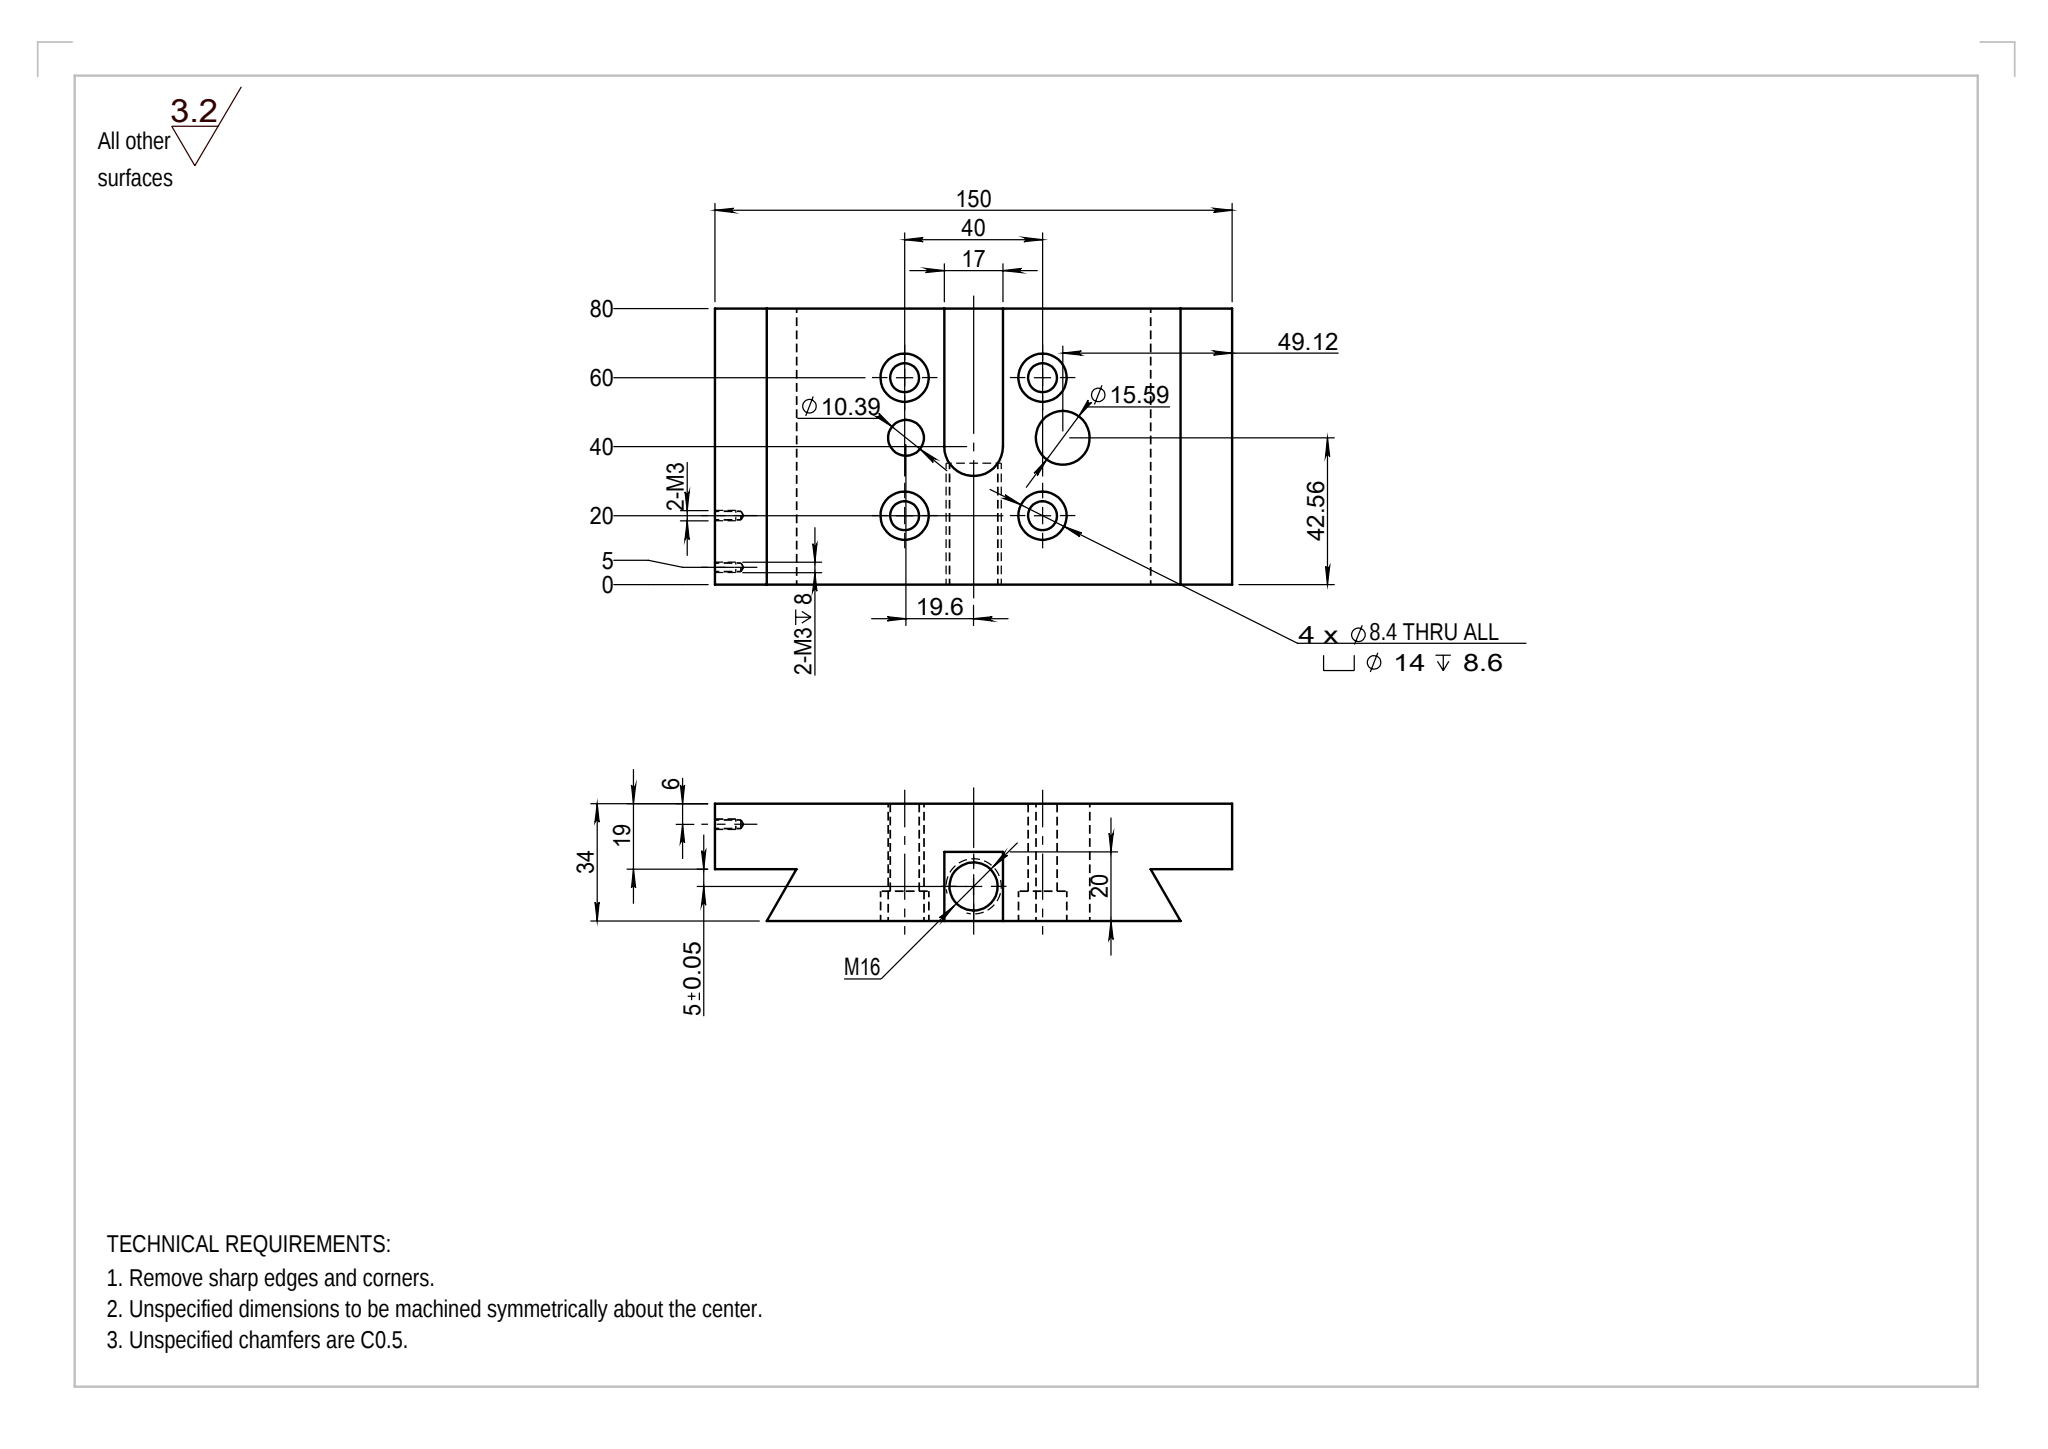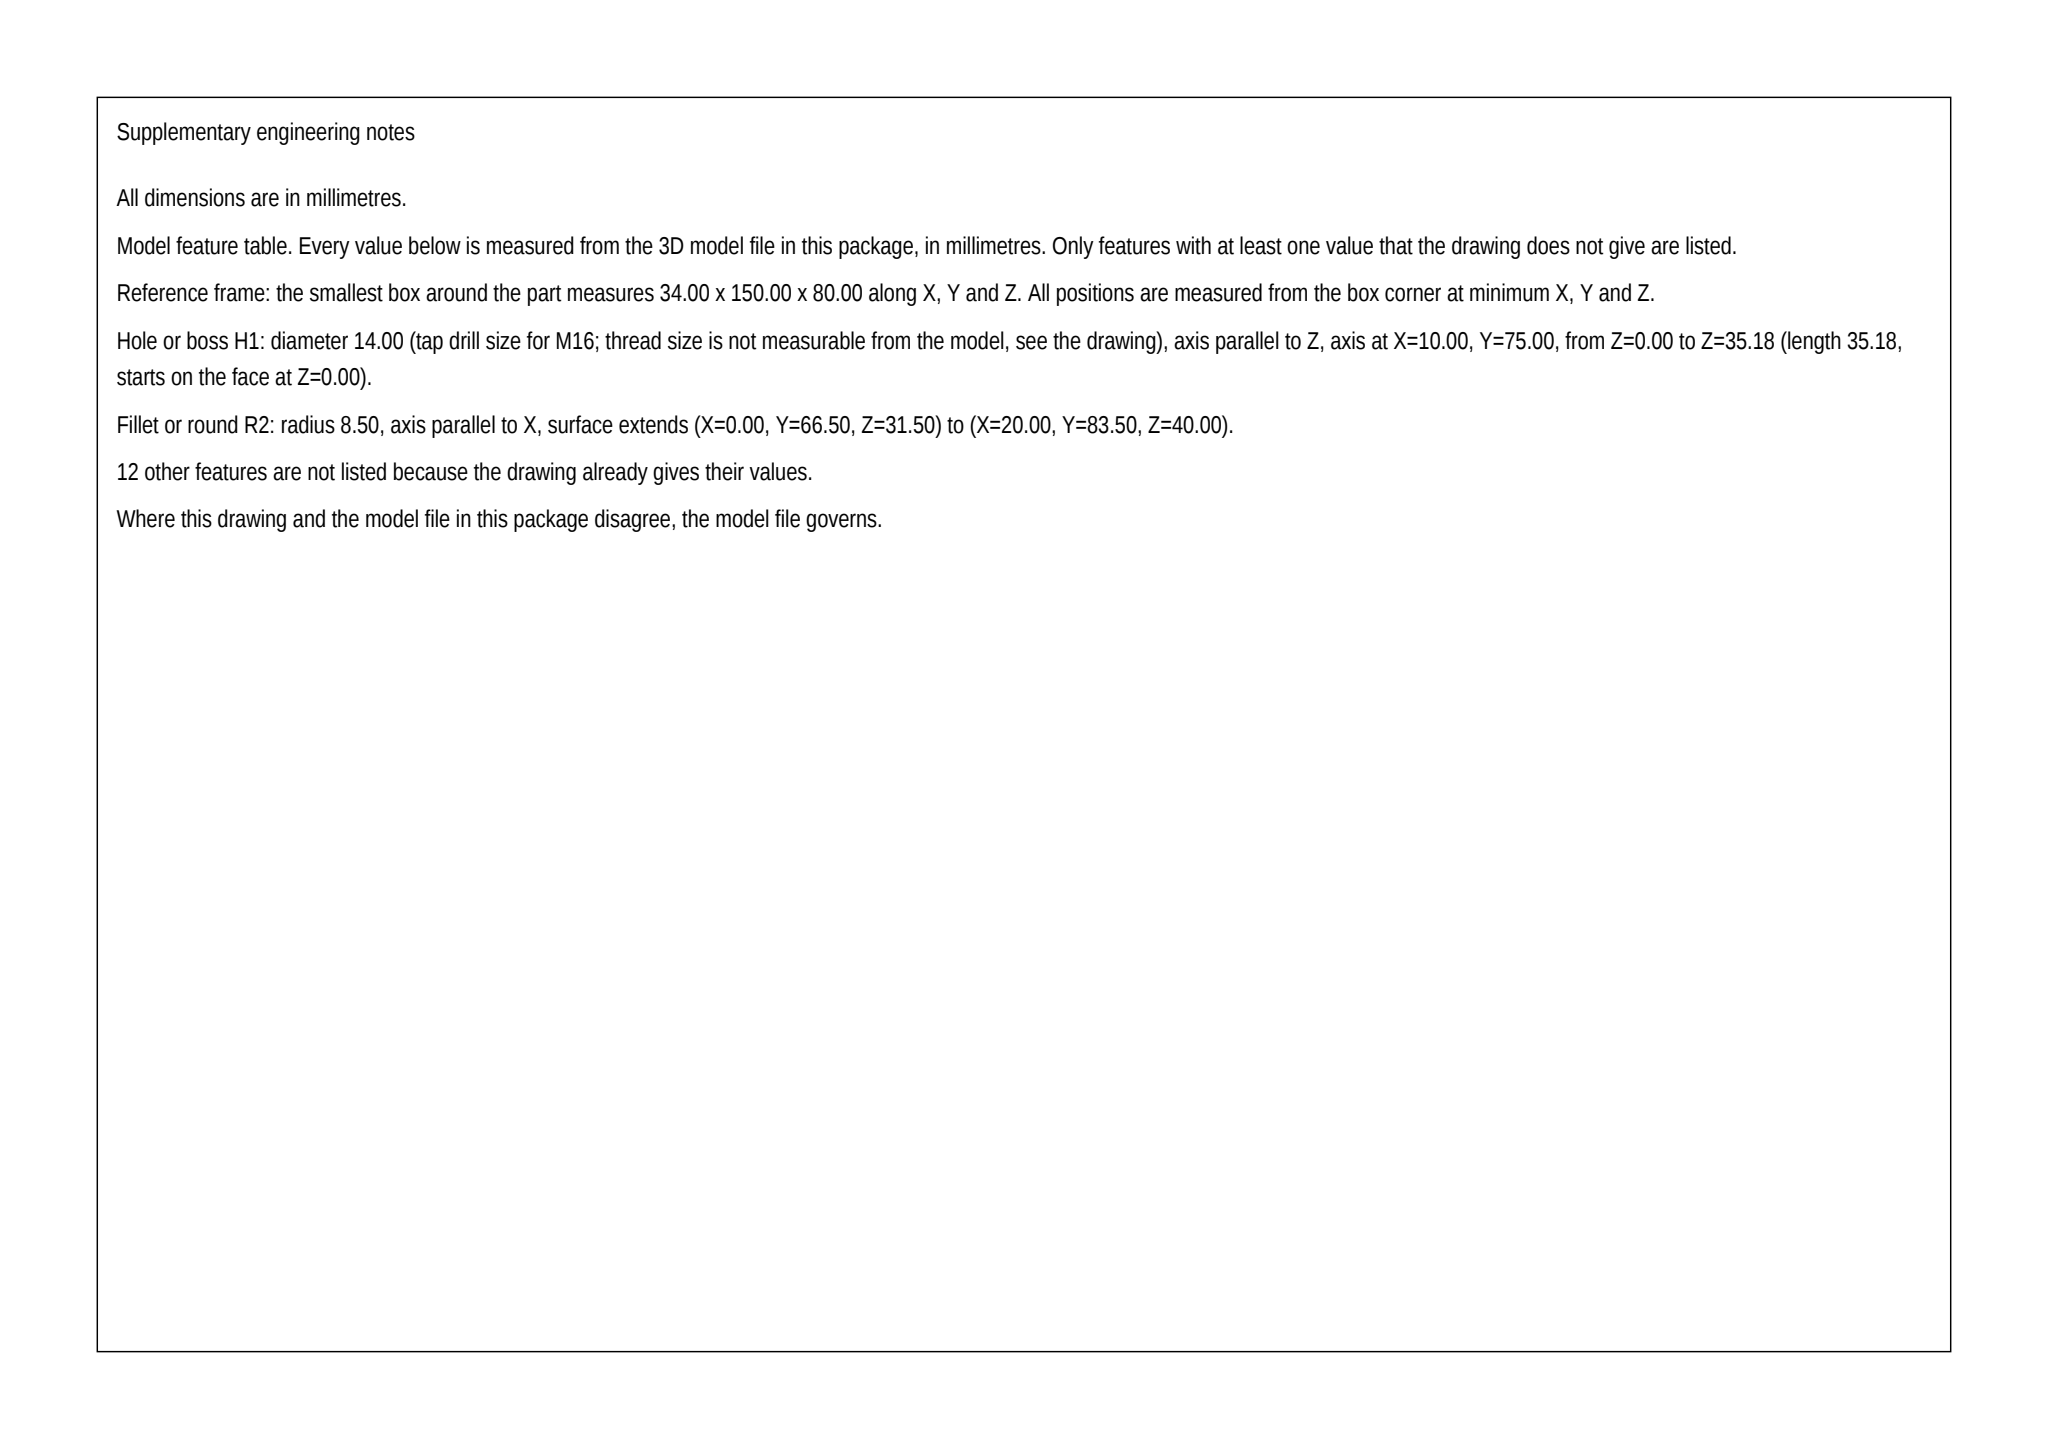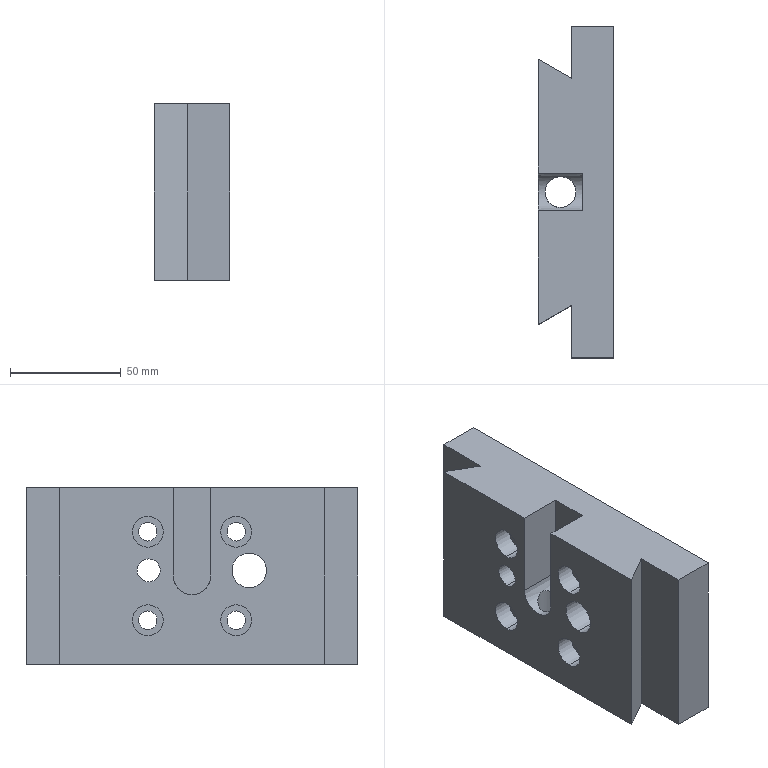Part | SolidWorks | mm | 1 solid | 48 faces | box 34 x 150 x 80 mm | volume 320387 mm3 | cylinder 27 | plane 17 | cone 4 | commonest cylinder face diameters 14 x10 8.4 x8 2.5 x4 15.591 x2 10.394 x2 17 x1
build123d program:
from build123d import *

# Parameters (mm, degrees)
SKETCH1_R                                       = 6
BOSS_EXTRUDE1_DEPTH                             = 80
CUT_EXTRUDE2_DEPTH                              = 20
M16_TAPPED_HOLE1_D                              = 14
M16_TAPPED_HOLE1_DEPTH                          = 56
M16_TAPPED_HOLE1_TIP                            = 4.206
M8_HEX_SOCKET_HEAD_CAP_SCREW_CBORE1_D           = 8.4
M8_HEX_SOCKET_HEAD_CAP_SCREW_CBORE1_CBORE_D     = 14
M8_HEX_SOCKET_HEAD_CAP_SCREW_CBORE1_CBORE_DEPTH = 8.6
M3_TAPPED_HOLE1_D                               = 2.5
M3_TAPPED_HOLE1_DEPTH                           = 7.5
M3_TAPPED_HOLE1_TIP                             = 0.7511
SKETCH10_R                                      = 7.796
SKETCH10_R_2                                    = 5.197
CUT_EXTRUDE4_DEPTH                              = 80


with BuildPart() as part:
    # Sketch1 → Boss-Extrude1 (new body)
    with BuildSketch(Plane.XY):
        Polygon((4, 75), (4, -75), (-15, -75), (-15, -51.34), (-30, -60), (-30, 60), (-15, 51.34), (-15, 75), align=None)
        with Locations((-20, 0)):
            Circle(SKETCH1_R, mode=Mode.SUBTRACT)
    extrude(amount=BOSS_EXTRUDE1_DEPTH)

    # Sketch3 → Cut-Extrude2 (cut)
    with BuildSketch(Plane.ZY.offset(30)):
        with BuildLine():
            Line((40, 8.5), (173.439, 8.5))
            ThreePointArc((173.439, 8.5), (181.939, 0), (173.439, -8.5))
            Line((173.439, -8.5), (40, -8.5))
            ThreePointArc((40, -8.5), (31.5, 0), (40, 8.5))
        make_face()
    extrude(amount=-CUT_EXTRUDE2_DEPTH, mode=Mode.SUBTRACT)

    # M16 Tapped Hole1
    with Locations(Plane(origin=(-20, 0, 0), x_dir=(-1, 0, 0), z_dir=(0, 0, -1))):
        with Locations((0, 0)):
            Hole(M16_TAPPED_HOLE1_D / 2, depth=M16_TAPPED_HOLE1_DEPTH)
            with Locations((0, 0, -(M16_TAPPED_HOLE1_DEPTH + M16_TAPPED_HOLE1_TIP / 2))):  # 118° drill point
                Cone(0, M16_TAPPED_HOLE1_D / 2, M16_TAPPED_HOLE1_TIP, mode=Mode.SUBTRACT)

    # M8 Hex Socket Head Cap Screw CBORE1 (through all)
    with Locations(Plane.ZY.offset(30)):
        with Locations((20, 20), (60, 20), (20, -20), (60, -20)):
            CounterBoreHole(M8_HEX_SOCKET_HEAD_CAP_SCREW_CBORE1_D / 2, M8_HEX_SOCKET_HEAD_CAP_SCREW_CBORE1_CBORE_D / 2, M8_HEX_SOCKET_HEAD_CAP_SCREW_CBORE1_CBORE_DEPTH)

    # M3 Tapped Hole1
    with Locations(Plane(origin=(0, 75, 0), x_dir=(1, 0, 0), z_dir=(0, 1, 0))):
        with Locations((-2, -5), (-2, -20)):
            Hole(M3_TAPPED_HOLE1_D / 2, depth=M3_TAPPED_HOLE1_DEPTH)
            with Locations((0, 0, -(M3_TAPPED_HOLE1_DEPTH + M3_TAPPED_HOLE1_TIP / 2))):  # 118° drill point
                Cone(0, M3_TAPPED_HOLE1_D / 2, M3_TAPPED_HOLE1_TIP, mode=Mode.SUBTRACT)

    # Sketch10 → Cut-Extrude4 (cut)
    with BuildSketch(Plane.ZY.offset(30)):
        with Locations((42.564, -25.877)):
            Circle(SKETCH10_R)
        with Locations((42.564, 19.597)):
            Circle(SKETCH10_R_2)
    extrude(amount=-CUT_EXTRUDE4_DEPTH, mode=Mode.SUBTRACT)


solid = part.part